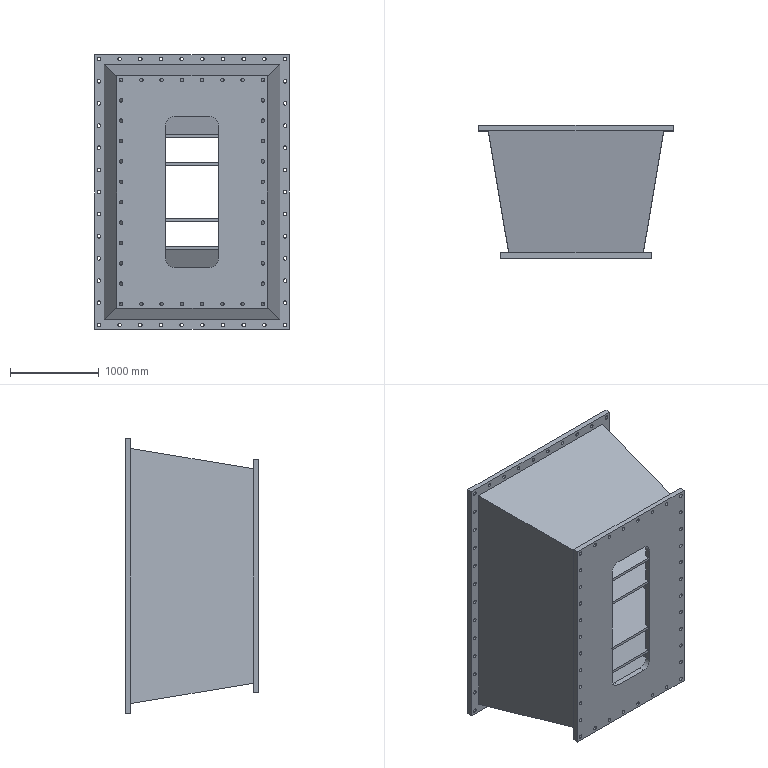Component | SolidWorks | RigidLegSaddleBody-2 | 1 solid | 230 faces | volume 1430372838 mm3 | cylinder 164 | plane 66 | commonest cylinder face diameters 40 x156 200 x8